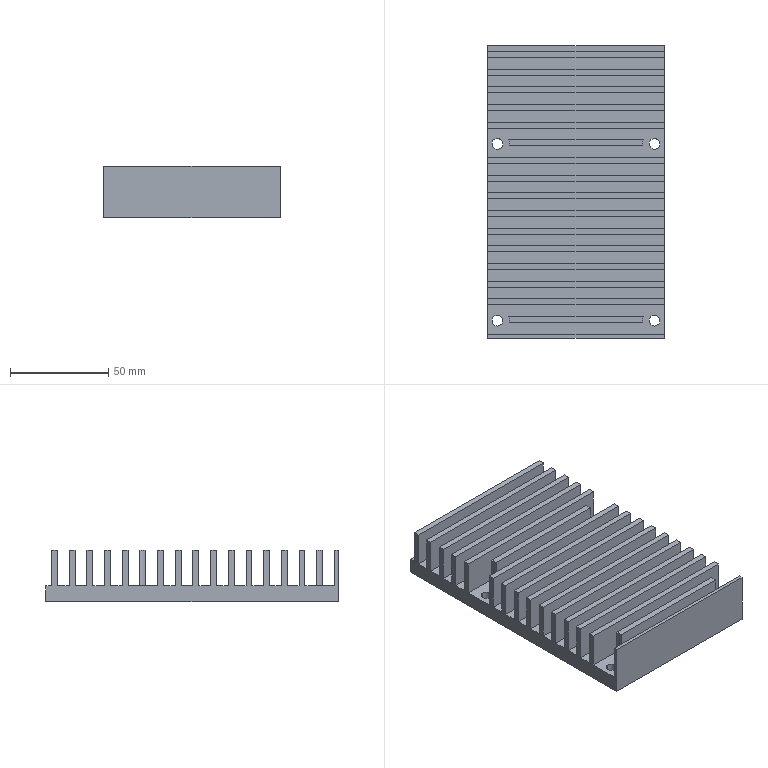CAM job | Mastercam | mm | 5 operations | part box 90 x 149 x 26
1. Contour (Ramp) | 9 - 10 平铣刀
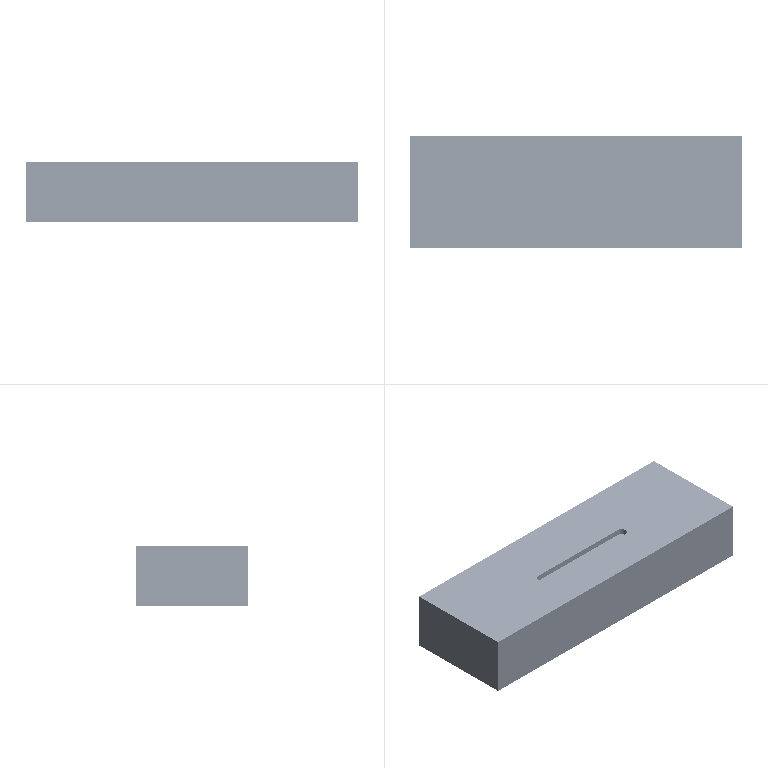2. Contour (2D) | 10 - 10 平铣刀
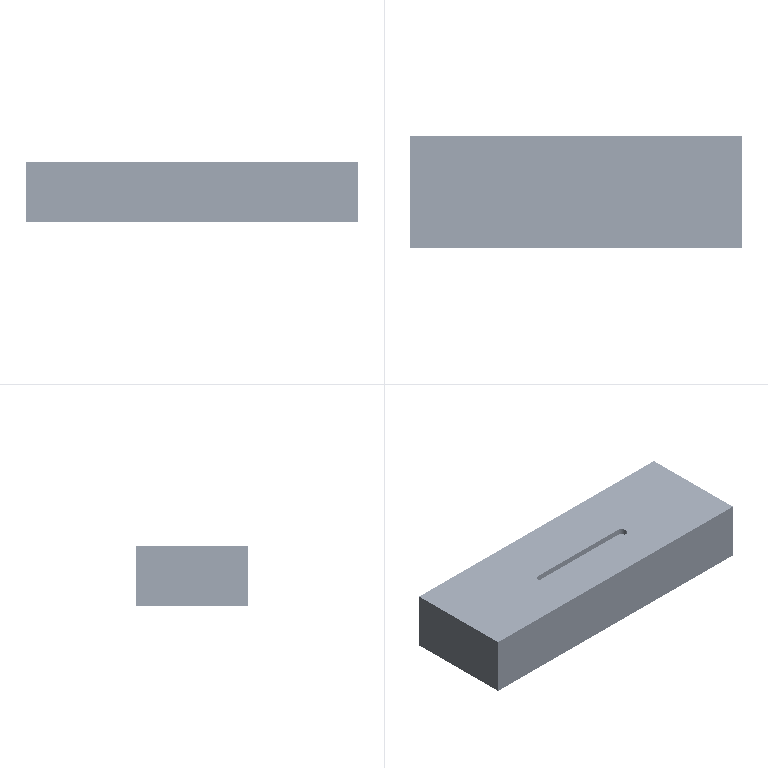3. Contour (Ramp) | 6 - 6 平铣刀
4. Drill/Counterbore | 5 - 4 倒角刀
5. Facing | 24 - 100 平铣刀